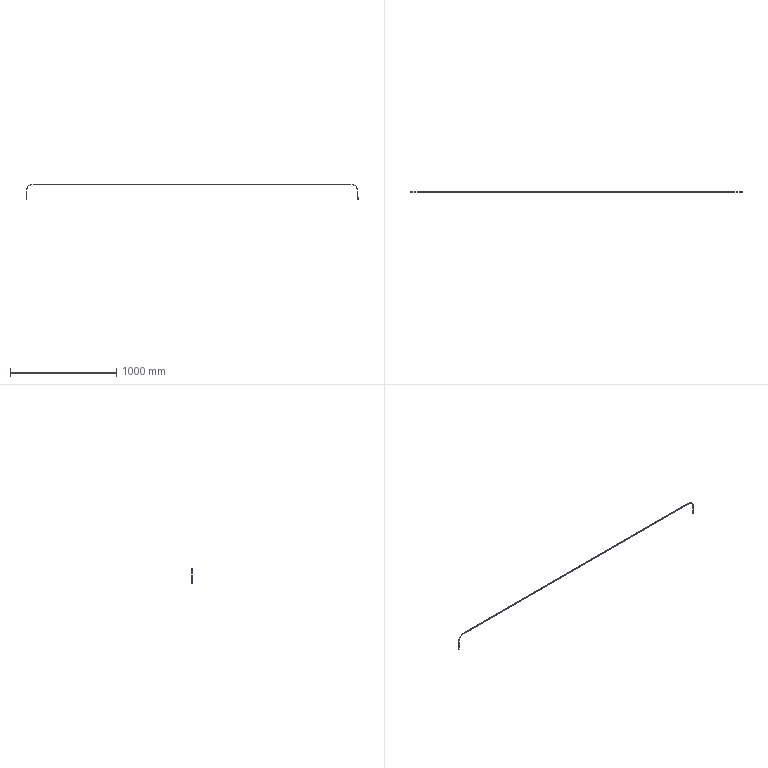Component | SolidWorks | A-SideAluminumCasingAssembly-1_A-SideSealant-1 | 1 solid | 22 faces | box 3131 x 6 x 149.5 mm | volume 60581 mm3 | plane 18 | cylinder 4 | commonest cylinder face diameters 139 x2 133 x2
STEP:
#1=COLOUR_RGB('',0.7922,0.8196,0.9333);
#2=FILL_AREA_STYLE_COLOUR('',#1);
#3=FILL_AREA_STYLE('',(#2));
#4=SURFACE_STYLE_FILL_AREA(#3);
#5=SURFACE_SIDE_STYLE('',(#4));
#6=SURFACE_STYLE_USAGE(.BOTH.,#5);
#7=PRESENTATION_STYLE_ASSIGNMENT((#6));
#8=CARTESIAN_POINT('',(80.551,91.024,73.819));
#9=VERTEX_POINT('',#8);
#10=CARTESIAN_POINT('',(80.551,91.024,73.937));
#11=VERTEX_POINT('',#10);
#12=CARTESIAN_POINT('',(80.551,91.024,73.937));
#13=DIRECTION('',(-0.,0.,1.));
#14=VECTOR('',#13,39.37);
#15=LINE('',#12,#14);
#16=EDGE_CURVE('',#9,#11,#15,.T.);
#17=ORIENTED_EDGE('',*,*,#16,.F.);
#18=CARTESIAN_POINT('',(-37.244,91.024,73.819));
#19=VERTEX_POINT('',#18);
#20=CARTESIAN_POINT('',(-37.244,91.024,73.819));
#21=DIRECTION('',(1.,0.,0.));
#22=VECTOR('',#21,39.37);
#23=LINE('',#20,#22);
#24=EDGE_CURVE('',#19,#9,#23,.T.);
#25=ORIENTED_EDGE('',*,*,#24,.F.);
#26=CARTESIAN_POINT('',(-37.244,91.024,73.937));
#27=VERTEX_POINT('',#26);
#28=CARTESIAN_POINT('',(-37.244,91.024,73.937));
#29=DIRECTION('',(-0.,0.,1.));
#30=VECTOR('',#29,39.37);
#31=LINE('',#28,#30);
#32=EDGE_CURVE('',#19,#27,#31,.T.);
#33=ORIENTED_EDGE('',*,*,#32,.T.);
#34=CARTESIAN_POINT('',(-37.244,91.024,73.937));
#35=DIRECTION('',(1.,0.,0.));
#36=VECTOR('',#35,39.37);
#37=LINE('',#34,#36);
#38=EDGE_CURVE('',#27,#11,#37,.T.);
#39=ORIENTED_EDGE('',*,*,#38,.T.);
#40=EDGE_LOOP('',(#17,#25,#33,#39));
#41=FACE_OUTER_BOUND('',#40,.T.);
#42=CARTESIAN_POINT('',(-37.244,91.024,73.937));
#43=DIRECTION('',(-0.,1.,-0.));
#44=DIRECTION('',(1.,0.,0.));
#45=AXIS2_PLACEMENT_3D('',#42,#43,#44);
#46=PLANE('',#45);
#47=ADVANCED_FACE('',(#41),#46,.T.);
#48=CARTESIAN_POINT('',(-37.244,90.787,73.819));
#49=VERTEX_POINT('',#48);
#50=CARTESIAN_POINT('',(-37.244,90.787,73.937));
#51=VERTEX_POINT('',#50);
#52=CARTESIAN_POINT('',(-37.244,90.787,73.937));
#53=DIRECTION('',(-0.,0.,1.));
#54=VECTOR('',#53,39.37);
#55=LINE('',#52,#54);
#56=EDGE_CURVE('',#49,#51,#55,.T.);
#57=ORIENTED_EDGE('',*,*,#56,.F.);
#58=CARTESIAN_POINT('',(80.551,90.787,73.819));
#59=VERTEX_POINT('',#58);
#60=CARTESIAN_POINT('',(-37.244,90.787,73.819));
#61=DIRECTION('',(1.,0.,0.));
#62=VECTOR('',#61,39.37);
#63=LINE('',#60,#62);
#64=EDGE_CURVE('',#49,#59,#63,.T.);
#65=ORIENTED_EDGE('',*,*,#64,.T.);
#66=CARTESIAN_POINT('',(80.551,90.787,73.937));
#67=VERTEX_POINT('',#66);
#68=CARTESIAN_POINT('',(80.551,90.787,73.937));
#69=DIRECTION('',(-0.,0.,1.));
#70=VECTOR('',#69,39.37);
#71=LINE('',#68,#70);
#72=EDGE_CURVE('',#59,#67,#71,.T.);
#73=ORIENTED_EDGE('',*,*,#72,.T.);
#74=CARTESIAN_POINT('',(-37.244,90.787,73.937));
#75=DIRECTION('',(1.,0.,0.));
#76=VECTOR('',#75,39.37);
#77=LINE('',#74,#76);
#78=EDGE_CURVE('',#51,#67,#77,.T.);
#79=ORIENTED_EDGE('',*,*,#78,.F.);
#80=EDGE_LOOP('',(#57,#65,#73,#79));
#81=FACE_OUTER_BOUND('',#80,.T.);
#82=CARTESIAN_POINT('',(-37.244,90.787,73.937));
#83=DIRECTION('',(-0.,1.,-0.));
#84=DIRECTION('',(1.,0.,0.));
#85=AXIS2_PLACEMENT_3D('',#82,#83,#84);
#86=PLANE('',#85);
#87=ADVANCED_FACE('',(#81),#86,.F.);
#88=ORIENTED_EDGE('',*,*,#78,.T.);
#89=CARTESIAN_POINT('',(80.551,91.024,73.937));
#90=DIRECTION('',(0.,-1.,0.));
#91=VECTOR('',#90,39.37);
#92=LINE('',#89,#91);
#93=EDGE_CURVE('',#11,#67,#92,.T.);
#94=ORIENTED_EDGE('',*,*,#93,.F.);
#95=ORIENTED_EDGE('',*,*,#38,.F.);
#96=CARTESIAN_POINT('',(-37.244,90.787,73.937));
#97=DIRECTION('',(-0.,1.,-0.));
#98=VECTOR('',#97,39.37);
#99=LINE('',#96,#98);
#100=EDGE_CURVE('',#51,#27,#99,.T.);
#101=ORIENTED_EDGE('',*,*,#100,.F.);
#102=EDGE_LOOP('',(#88,#94,#95,#101));
#103=FACE_OUTER_BOUND('',#102,.T.);
#104=CARTESIAN_POINT('',(-37.244,90.787,73.937));
#105=DIRECTION('',(0.,-0.,-1.));
#106=DIRECTION('',(-0.,1.,-0.));
#107=AXIS2_PLACEMENT_3D('',#104,#105,#106);
#108=PLANE('',#107);
#109=ADVANCED_FACE('',(#103),#108,.F.);
#110=ORIENTED_EDGE('',*,*,#64,.F.);
#111=CARTESIAN_POINT('',(-37.244,90.787,73.819));
#112=DIRECTION('',(-0.,1.,-0.));
#113=VECTOR('',#112,39.37);
#114=LINE('',#111,#113);
#115=EDGE_CURVE('',#49,#19,#114,.T.);
#116=ORIENTED_EDGE('',*,*,#115,.T.);
#117=ORIENTED_EDGE('',*,*,#24,.T.);
#118=CARTESIAN_POINT('',(80.551,90.787,73.819));
#119=DIRECTION('',(0.,-1.,0.));
#120=VECTOR('',#119,39.37);
#121=LINE('',#118,#120);
#122=EDGE_CURVE('',#9,#59,#121,.T.);
#123=ORIENTED_EDGE('',*,*,#122,.T.);
#124=EDGE_LOOP('',(#110,#116,#117,#123));
#125=FACE_OUTER_BOUND('',#124,.T.);
#126=CARTESIAN_POINT('',(-37.244,90.787,73.819));
#127=DIRECTION('',(0.,-0.,-1.));
#128=DIRECTION('',(-0.,1.,-0.));
#129=AXIS2_PLACEMENT_3D('',#126,#127,#128);
#130=PLANE('',#129);
#131=ADVANCED_FACE('',(#125),#130,.T.);
#132=CARTESIAN_POINT('',(-39.862,90.787,71.201));
#133=VERTEX_POINT('',#132);
#134=CARTESIAN_POINT('',(-39.98,90.787,71.201));
#135=VERTEX_POINT('',#134);
#136=CARTESIAN_POINT('',(-39.98,90.787,71.201));
#137=DIRECTION('',(-1.,-0.,0.));
#138=VECTOR('',#137,39.37);
#139=LINE('',#136,#138);
#140=EDGE_CURVE('',#133,#135,#139,.T.);
#141=ORIENTED_EDGE('',*,*,#140,.F.);
#142=CARTESIAN_POINT('',(-37.244,90.787,71.201));
#143=DIRECTION('',(0.,-1.,0.));
#144=DIRECTION('',(0.,0.,1.));
#145=AXIS2_PLACEMENT_3D('',#142,#143,#144);
#146=CIRCLE('',#145,2.618);
#147=EDGE_CURVE('',#49,#133,#146,.T.);
#148=ORIENTED_EDGE('',*,*,#147,.F.);
#149=ORIENTED_EDGE('',*,*,#56,.T.);
#150=CARTESIAN_POINT('',(-37.244,90.787,71.201));
#151=DIRECTION('',(0.,-1.,0.));
#152=DIRECTION('',(0.,0.,1.));
#153=AXIS2_PLACEMENT_3D('',#150,#151,#152);
#154=CIRCLE('',#153,2.736);
#155=EDGE_CURVE('',#51,#135,#154,.T.);
#156=ORIENTED_EDGE('',*,*,#155,.T.);
#157=EDGE_LOOP('',(#141,#148,#149,#156));
#158=FACE_OUTER_BOUND('',#157,.T.);
#159=CARTESIAN_POINT('',(-37.244,90.787,71.201));
#160=DIRECTION('',(0.,-1.,0.));
#161=DIRECTION('',(0.,-0.,-1.));
#162=AXIS2_PLACEMENT_3D('',#159,#160,#161);
#163=PLANE('',#162);
#164=ADVANCED_FACE('',(#158),#163,.T.);
#165=CARTESIAN_POINT('',(-39.862,91.024,71.201));
#166=VERTEX_POINT('',#165);
#167=CARTESIAN_POINT('',(-37.244,91.024,71.201));
#168=DIRECTION('',(-0.,1.,-0.));
#169=DIRECTION('',(0.,0.,1.));
#170=AXIS2_PLACEMENT_3D('',#167,#168,#169);
#171=CIRCLE('',#170,2.618);
#172=EDGE_CURVE('',#166,#19,#171,.T.);
#173=ORIENTED_EDGE('',*,*,#172,.F.);
#174=CARTESIAN_POINT('',(-39.98,91.024,71.201));
#175=VERTEX_POINT('',#174);
#176=CARTESIAN_POINT('',(-39.862,91.024,71.201));
#177=DIRECTION('',(-1.,-0.,0.));
#178=VECTOR('',#177,39.37);
#179=LINE('',#176,#178);
#180=EDGE_CURVE('',#166,#175,#179,.T.);
#181=ORIENTED_EDGE('',*,*,#180,.T.);
#182=CARTESIAN_POINT('',(-37.244,91.024,71.201));
#183=DIRECTION('',(-0.,1.,-0.));
#184=DIRECTION('',(0.,0.,1.));
#185=AXIS2_PLACEMENT_3D('',#182,#183,#184);
#186=CIRCLE('',#185,2.736);
#187=EDGE_CURVE('',#175,#27,#186,.T.);
#188=ORIENTED_EDGE('',*,*,#187,.T.);
#189=ORIENTED_EDGE('',*,*,#32,.F.);
#190=EDGE_LOOP('',(#173,#181,#188,#189));
#191=FACE_OUTER_BOUND('',#190,.T.);
#192=CARTESIAN_POINT('',(-37.244,91.024,71.201));
#193=DIRECTION('',(0.,-1.,0.));
#194=DIRECTION('',(0.,-0.,-1.));
#195=AXIS2_PLACEMENT_3D('',#192,#193,#194);
#196=PLANE('',#195);
#197=ADVANCED_FACE('',(#191),#196,.F.);
#198=ORIENTED_EDGE('',*,*,#100,.T.);
#199=ORIENTED_EDGE('',*,*,#187,.F.);
#200=CARTESIAN_POINT('',(-39.98,90.787,71.201));
#201=DIRECTION('',(0.,-1.,0.));
#202=VECTOR('',#201,39.37);
#203=LINE('',#200,#202);
#204=EDGE_CURVE('',#175,#135,#203,.T.);
#205=ORIENTED_EDGE('',*,*,#204,.T.);
#206=ORIENTED_EDGE('',*,*,#155,.F.);
#207=EDGE_LOOP('',(#198,#199,#205,#206));
#208=FACE_OUTER_BOUND('',#207,.T.);
#209=CARTESIAN_POINT('',(-37.244,91.024,71.201));
#210=DIRECTION('',(-0.,1.,-0.));
#211=DIRECTION('',(-1.,-0.,0.));
#212=AXIS2_PLACEMENT_3D('',#209,#210,#211);
#213=CYLINDRICAL_SURFACE('',#212,2.736);
#214=ADVANCED_FACE('',(#208),#213,.T.);
#215=ORIENTED_EDGE('',*,*,#115,.F.);
#216=ORIENTED_EDGE('',*,*,#147,.T.);
#217=CARTESIAN_POINT('',(-39.862,90.787,71.201));
#218=DIRECTION('',(-0.,1.,-0.));
#219=VECTOR('',#218,39.37);
#220=LINE('',#217,#219);
#221=EDGE_CURVE('',#133,#166,#220,.T.);
#222=ORIENTED_EDGE('',*,*,#221,.T.);
#223=ORIENTED_EDGE('',*,*,#172,.T.);
#224=EDGE_LOOP('',(#215,#216,#222,#223));
#225=FACE_OUTER_BOUND('',#224,.T.);
#226=CARTESIAN_POINT('',(-37.244,91.024,71.201));
#227=DIRECTION('',(-0.,1.,-0.));
#228=DIRECTION('',(-1.,-0.,0.));
#229=AXIS2_PLACEMENT_3D('',#226,#227,#228);
#230=CYLINDRICAL_SURFACE('',#229,2.618);
#231=ADVANCED_FACE('',(#225),#230,.F.);
#232=ORIENTED_EDGE('',*,*,#140,.T.);
#233=CARTESIAN_POINT('',(-39.98,90.787,68.051));
#234=VERTEX_POINT('',#233);
#235=CARTESIAN_POINT('',(-39.98,90.787,73.819));
#236=DIRECTION('',(0.,0.,1.));
#237=VECTOR('',#236,39.37);
#238=LINE('',#235,#237);
#239=EDGE_CURVE('',#234,#135,#238,.T.);
#240=ORIENTED_EDGE('',*,*,#239,.F.);
#241=CARTESIAN_POINT('',(-39.862,90.787,68.051));
#242=VERTEX_POINT('',#241);
#243=CARTESIAN_POINT('',(-39.98,90.787,68.051));
#244=DIRECTION('',(1.,0.,-0.));
#245=VECTOR('',#244,39.37);
#246=LINE('',#243,#245);
#247=EDGE_CURVE('',#234,#242,#246,.T.);
#248=ORIENTED_EDGE('',*,*,#247,.T.);
#249=CARTESIAN_POINT('',(-39.862,90.787,73.819));
#250=DIRECTION('',(0.,0.,1.));
#251=VECTOR('',#250,39.37);
#252=LINE('',#249,#251);
#253=EDGE_CURVE('',#242,#133,#252,.T.);
#254=ORIENTED_EDGE('',*,*,#253,.T.);
#255=EDGE_LOOP('',(#232,#240,#248,#254));
#256=FACE_OUTER_BOUND('',#255,.T.);
#257=CARTESIAN_POINT('',(-39.98,90.787,73.819));
#258=DIRECTION('',(-0.,1.,-0.));
#259=DIRECTION('',(-0.,0.,1.));
#260=AXIS2_PLACEMENT_3D('',#257,#258,#259);
#261=PLANE('',#260);
#262=ADVANCED_FACE('',(#256),#261,.F.);
#263=ORIENTED_EDGE('',*,*,#180,.F.);
#264=CARTESIAN_POINT('',(-39.862,91.024,68.051));
#265=VERTEX_POINT('',#264);
#266=CARTESIAN_POINT('',(-39.862,91.024,68.051));
#267=DIRECTION('',(-0.,-0.,-1.));
#268=VECTOR('',#267,39.37);
#269=LINE('',#266,#268);
#270=EDGE_CURVE('',#166,#265,#269,.T.);
#271=ORIENTED_EDGE('',*,*,#270,.T.);
#272=CARTESIAN_POINT('',(-39.98,91.024,68.051));
#273=VERTEX_POINT('',#272);
#274=CARTESIAN_POINT('',(-39.98,91.024,68.051));
#275=DIRECTION('',(1.,0.,-0.));
#276=VECTOR('',#275,39.37);
#277=LINE('',#274,#276);
#278=EDGE_CURVE('',#273,#265,#277,.T.);
#279=ORIENTED_EDGE('',*,*,#278,.F.);
#280=CARTESIAN_POINT('',(-39.98,91.024,73.819));
#281=DIRECTION('',(-0.,-0.,-1.));
#282=VECTOR('',#281,39.37);
#283=LINE('',#280,#282);
#284=EDGE_CURVE('',#175,#273,#283,.T.);
#285=ORIENTED_EDGE('',*,*,#284,.F.);
#286=EDGE_LOOP('',(#263,#271,#279,#285));
#287=FACE_OUTER_BOUND('',#286,.T.);
#288=CARTESIAN_POINT('',(-39.98,91.024,68.051));
#289=DIRECTION('',(0.,-1.,0.));
#290=DIRECTION('',(0.,-0.,-1.));
#291=AXIS2_PLACEMENT_3D('',#288,#289,#290);
#292=PLANE('',#291);
#293=ADVANCED_FACE('',(#287),#292,.F.);
#294=ORIENTED_EDGE('',*,*,#204,.F.);
#295=ORIENTED_EDGE('',*,*,#284,.T.);
#296=CARTESIAN_POINT('',(-39.98,90.787,68.051));
#297=DIRECTION('',(0.,-1.,0.));
#298=VECTOR('',#297,39.37);
#299=LINE('',#296,#298);
#300=EDGE_CURVE('',#273,#234,#299,.T.);
#301=ORIENTED_EDGE('',*,*,#300,.T.);
#302=ORIENTED_EDGE('',*,*,#239,.T.);
#303=EDGE_LOOP('',(#294,#295,#301,#302));
#304=FACE_OUTER_BOUND('',#303,.T.);
#305=CARTESIAN_POINT('',(-39.98,90.787,73.819));
#306=DIRECTION('',(1.,0.,-0.));
#307=DIRECTION('',(0.,0.,1.));
#308=AXIS2_PLACEMENT_3D('',#305,#306,#307);
#309=PLANE('',#308);
#310=ADVANCED_FACE('',(#304),#309,.F.);
#311=ORIENTED_EDGE('',*,*,#270,.F.);
#312=ORIENTED_EDGE('',*,*,#221,.F.);
#313=ORIENTED_EDGE('',*,*,#253,.F.);
#314=CARTESIAN_POINT('',(-39.862,90.787,68.051));
#315=DIRECTION('',(0.,-1.,0.));
#316=VECTOR('',#315,39.37);
#317=LINE('',#314,#316);
#318=EDGE_CURVE('',#265,#242,#317,.T.);
#319=ORIENTED_EDGE('',*,*,#318,.F.);
#320=EDGE_LOOP('',(#311,#312,#313,#319));
#321=FACE_OUTER_BOUND('',#320,.T.);
#322=CARTESIAN_POINT('',(-39.862,90.787,73.819));
#323=DIRECTION('',(1.,0.,-0.));
#324=DIRECTION('',(0.,0.,1.));
#325=AXIS2_PLACEMENT_3D('',#322,#323,#324);
#326=PLANE('',#325);
#327=ADVANCED_FACE('',(#321),#326,.T.);
#328=ORIENTED_EDGE('',*,*,#318,.T.);
#329=ORIENTED_EDGE('',*,*,#247,.F.);
#330=ORIENTED_EDGE('',*,*,#300,.F.);
#331=ORIENTED_EDGE('',*,*,#278,.T.);
#332=EDGE_LOOP('',(#328,#329,#330,#331));
#333=FACE_OUTER_BOUND('',#332,.T.);
#334=CARTESIAN_POINT('',(-39.98,90.787,68.051));
#335=DIRECTION('',(0.,0.,1.));
#336=DIRECTION('',(-1.,-0.,0.));
#337=AXIS2_PLACEMENT_3D('',#334,#335,#336);
#338=PLANE('',#337);
#339=ADVANCED_FACE('',(#333),#338,.F.);
#340=CARTESIAN_POINT('',(83.169,91.024,71.201));
#341=VERTEX_POINT('',#340);
#342=CARTESIAN_POINT('',(83.287,91.024,71.201));
#343=VERTEX_POINT('',#342);
#344=CARTESIAN_POINT('',(83.287,91.024,71.201));
#345=DIRECTION('',(1.,0.,0.));
#346=VECTOR('',#345,39.37);
#347=LINE('',#344,#346);
#348=EDGE_CURVE('',#341,#343,#347,.T.);
#349=ORIENTED_EDGE('',*,*,#348,.F.);
#350=CARTESIAN_POINT('',(80.551,91.024,71.201));
#351=DIRECTION('',(-0.,1.,-0.));
#352=DIRECTION('',(0.,-0.,-1.));
#353=AXIS2_PLACEMENT_3D('',#350,#351,#352);
#354=CIRCLE('',#353,2.618);
#355=EDGE_CURVE('',#9,#341,#354,.T.);
#356=ORIENTED_EDGE('',*,*,#355,.F.);
#357=ORIENTED_EDGE('',*,*,#16,.T.);
#358=CARTESIAN_POINT('',(80.551,91.024,71.201));
#359=DIRECTION('',(-0.,1.,-0.));
#360=DIRECTION('',(0.,-0.,-1.));
#361=AXIS2_PLACEMENT_3D('',#358,#359,#360);
#362=CIRCLE('',#361,2.736);
#363=EDGE_CURVE('',#11,#343,#362,.T.);
#364=ORIENTED_EDGE('',*,*,#363,.T.);
#365=EDGE_LOOP('',(#349,#356,#357,#364));
#366=FACE_OUTER_BOUND('',#365,.T.);
#367=CARTESIAN_POINT('',(80.551,91.024,71.201));
#368=DIRECTION('',(-0.,1.,-0.));
#369=DIRECTION('',(-0.,0.,1.));
#370=AXIS2_PLACEMENT_3D('',#367,#368,#369);
#371=PLANE('',#370);
#372=ADVANCED_FACE('',(#366),#371,.T.);
#373=CARTESIAN_POINT('',(83.169,90.787,71.201));
#374=VERTEX_POINT('',#373);
#375=CARTESIAN_POINT('',(80.551,90.787,71.201));
#376=DIRECTION('',(0.,-1.,0.));
#377=DIRECTION('',(0.,-0.,-1.));
#378=AXIS2_PLACEMENT_3D('',#375,#376,#377);
#379=CIRCLE('',#378,2.618);
#380=EDGE_CURVE('',#374,#59,#379,.T.);
#381=ORIENTED_EDGE('',*,*,#380,.F.);
#382=CARTESIAN_POINT('',(83.287,90.787,71.201));
#383=VERTEX_POINT('',#382);
#384=CARTESIAN_POINT('',(83.169,90.787,71.201));
#385=DIRECTION('',(1.,0.,0.));
#386=VECTOR('',#385,39.37);
#387=LINE('',#384,#386);
#388=EDGE_CURVE('',#374,#383,#387,.T.);
#389=ORIENTED_EDGE('',*,*,#388,.T.);
#390=CARTESIAN_POINT('',(80.551,90.787,71.201));
#391=DIRECTION('',(0.,-1.,0.));
#392=DIRECTION('',(0.,-0.,-1.));
#393=AXIS2_PLACEMENT_3D('',#390,#391,#392);
#394=CIRCLE('',#393,2.736);
#395=EDGE_CURVE('',#383,#67,#394,.T.);
#396=ORIENTED_EDGE('',*,*,#395,.T.);
#397=ORIENTED_EDGE('',*,*,#72,.F.);
#398=EDGE_LOOP('',(#381,#389,#396,#397));
#399=FACE_OUTER_BOUND('',#398,.T.);
#400=CARTESIAN_POINT('',(80.551,90.787,71.201));
#401=DIRECTION('',(-0.,1.,-0.));
#402=DIRECTION('',(-0.,0.,1.));
#403=AXIS2_PLACEMENT_3D('',#400,#401,#402);
#404=PLANE('',#403);
#405=ADVANCED_FACE('',(#399),#404,.F.);
#406=ORIENTED_EDGE('',*,*,#93,.T.);
#407=ORIENTED_EDGE('',*,*,#395,.F.);
#408=CARTESIAN_POINT('',(83.287,91.024,71.201));
#409=DIRECTION('',(-0.,1.,-0.));
#410=VECTOR('',#409,39.37);
#411=LINE('',#408,#410);
#412=EDGE_CURVE('',#383,#343,#411,.T.);
#413=ORIENTED_EDGE('',*,*,#412,.T.);
#414=ORIENTED_EDGE('',*,*,#363,.F.);
#415=EDGE_LOOP('',(#406,#407,#413,#414));
#416=FACE_OUTER_BOUND('',#415,.T.);
#417=CARTESIAN_POINT('',(80.551,90.787,71.201));
#418=DIRECTION('',(0.,-1.,0.));
#419=DIRECTION('',(1.,0.,0.));
#420=AXIS2_PLACEMENT_3D('',#417,#418,#419);
#421=CYLINDRICAL_SURFACE('',#420,2.736);
#422=ADVANCED_FACE('',(#416),#421,.T.);
#423=ORIENTED_EDGE('',*,*,#122,.F.);
#424=ORIENTED_EDGE('',*,*,#355,.T.);
#425=CARTESIAN_POINT('',(83.169,91.024,71.201));
#426=DIRECTION('',(0.,-1.,0.));
#427=VECTOR('',#426,39.37);
#428=LINE('',#425,#427);
#429=EDGE_CURVE('',#341,#374,#428,.T.);
#430=ORIENTED_EDGE('',*,*,#429,.T.);
#431=ORIENTED_EDGE('',*,*,#380,.T.);
#432=EDGE_LOOP('',(#423,#424,#430,#431));
#433=FACE_OUTER_BOUND('',#432,.T.);
#434=CARTESIAN_POINT('',(80.551,90.787,71.201));
#435=DIRECTION('',(0.,-1.,0.));
#436=DIRECTION('',(1.,0.,0.));
#437=AXIS2_PLACEMENT_3D('',#434,#435,#436);
#438=CYLINDRICAL_SURFACE('',#437,2.618);
#439=ADVANCED_FACE('',(#433),#438,.F.);
#440=ORIENTED_EDGE('',*,*,#348,.T.);
#441=CARTESIAN_POINT('',(83.287,91.024,68.051));
#442=VERTEX_POINT('',#441);
#443=CARTESIAN_POINT('',(83.287,91.024,73.819));
#444=DIRECTION('',(-0.,0.,1.));
#445=VECTOR('',#444,39.37);
#446=LINE('',#443,#445);
#447=EDGE_CURVE('',#442,#343,#446,.T.);
#448=ORIENTED_EDGE('',*,*,#447,.F.);
#449=CARTESIAN_POINT('',(83.169,91.024,68.051));
#450=VERTEX_POINT('',#449);
#451=CARTESIAN_POINT('',(83.287,91.024,68.051));
#452=DIRECTION('',(-1.,-0.,-0.));
#453=VECTOR('',#452,39.37);
#454=LINE('',#451,#453);
#455=EDGE_CURVE('',#442,#450,#454,.T.);
#456=ORIENTED_EDGE('',*,*,#455,.T.);
#457=CARTESIAN_POINT('',(83.169,91.024,73.819));
#458=DIRECTION('',(-0.,0.,1.));
#459=VECTOR('',#458,39.37);
#460=LINE('',#457,#459);
#461=EDGE_CURVE('',#450,#341,#460,.T.);
#462=ORIENTED_EDGE('',*,*,#461,.T.);
#463=EDGE_LOOP('',(#440,#448,#456,#462));
#464=FACE_OUTER_BOUND('',#463,.T.);
#465=CARTESIAN_POINT('',(83.287,91.024,73.819));
#466=DIRECTION('',(0.,-1.,0.));
#467=DIRECTION('',(0.,-0.,-1.));
#468=AXIS2_PLACEMENT_3D('',#465,#466,#467);
#469=PLANE('',#468);
#470=ADVANCED_FACE('',(#464),#469,.F.);
#471=ORIENTED_EDGE('',*,*,#388,.F.);
#472=CARTESIAN_POINT('',(83.169,90.787,68.051));
#473=VERTEX_POINT('',#472);
#474=CARTESIAN_POINT('',(83.169,90.787,68.051));
#475=DIRECTION('',(0.,-0.,-1.));
#476=VECTOR('',#475,39.37);
#477=LINE('',#474,#476);
#478=EDGE_CURVE('',#374,#473,#477,.T.);
#479=ORIENTED_EDGE('',*,*,#478,.T.);
#480=CARTESIAN_POINT('',(83.287,90.787,68.051));
#481=VERTEX_POINT('',#480);
#482=CARTESIAN_POINT('',(83.287,90.787,68.051));
#483=DIRECTION('',(-1.,-0.,-0.));
#484=VECTOR('',#483,39.37);
#485=LINE('',#482,#484);
#486=EDGE_CURVE('',#481,#473,#485,.T.);
#487=ORIENTED_EDGE('',*,*,#486,.F.);
#488=CARTESIAN_POINT('',(83.287,90.787,73.819));
#489=DIRECTION('',(0.,-0.,-1.));
#490=VECTOR('',#489,39.37);
#491=LINE('',#488,#490);
#492=EDGE_CURVE('',#383,#481,#491,.T.);
#493=ORIENTED_EDGE('',*,*,#492,.F.);
#494=EDGE_LOOP('',(#471,#479,#487,#493));
#495=FACE_OUTER_BOUND('',#494,.T.);
#496=CARTESIAN_POINT('',(83.287,90.787,68.051));
#497=DIRECTION('',(-0.,1.,-0.));
#498=DIRECTION('',(-0.,0.,1.));
#499=AXIS2_PLACEMENT_3D('',#496,#497,#498);
#500=PLANE('',#499);
#501=ADVANCED_FACE('',(#495),#500,.F.);
#502=ORIENTED_EDGE('',*,*,#412,.F.);
#503=ORIENTED_EDGE('',*,*,#492,.T.);
#504=CARTESIAN_POINT('',(83.287,90.787,68.051));
#505=DIRECTION('',(-0.,1.,-0.));
#506=VECTOR('',#505,39.37);
#507=LINE('',#504,#506);
#508=EDGE_CURVE('',#481,#442,#507,.T.);
#509=ORIENTED_EDGE('',*,*,#508,.T.);
#510=ORIENTED_EDGE('',*,*,#447,.T.);
#511=EDGE_LOOP('',(#502,#503,#509,#510));
#512=FACE_OUTER_BOUND('',#511,.T.);
#513=CARTESIAN_POINT('',(83.287,90.787,73.819));
#514=DIRECTION('',(-1.,-0.,-0.));
#515=DIRECTION('',(0.,-0.,-1.));
#516=AXIS2_PLACEMENT_3D('',#513,#514,#515);
#517=PLANE('',#516);
#518=ADVANCED_FACE('',(#512),#517,.F.);
#519=ORIENTED_EDGE('',*,*,#478,.F.);
#520=ORIENTED_EDGE('',*,*,#429,.F.);
#521=ORIENTED_EDGE('',*,*,#461,.F.);
#522=CARTESIAN_POINT('',(83.169,91.024,68.051));
#523=DIRECTION('',(-0.,1.,-0.));
#524=VECTOR('',#523,39.37);
#525=LINE('',#522,#524);
#526=EDGE_CURVE('',#473,#450,#525,.T.);
#527=ORIENTED_EDGE('',*,*,#526,.F.);
#528=EDGE_LOOP('',(#519,#520,#521,#527));
#529=FACE_OUTER_BOUND('',#528,.T.);
#530=CARTESIAN_POINT('',(83.169,90.787,73.819));
#531=DIRECTION('',(-1.,-0.,-0.));
#532=DIRECTION('',(0.,-0.,-1.));
#533=AXIS2_PLACEMENT_3D('',#530,#531,#532);
#534=PLANE('',#533);
#535=ADVANCED_FACE('',(#529),#534,.T.);
#536=ORIENTED_EDGE('',*,*,#526,.T.);
#537=ORIENTED_EDGE('',*,*,#455,.F.);
#538=ORIENTED_EDGE('',*,*,#508,.F.);
#539=ORIENTED_EDGE('',*,*,#486,.T.);
#540=EDGE_LOOP('',(#536,#537,#538,#539));
#541=FACE_OUTER_BOUND('',#540,.T.);
#542=CARTESIAN_POINT('',(83.287,91.024,68.051));
#543=DIRECTION('',(-0.,0.,1.));
#544=DIRECTION('',(-1.,-0.,-0.));
#545=AXIS2_PLACEMENT_3D('',#542,#543,#544);
#546=PLANE('',#545);
#547=ADVANCED_FACE('',(#541),#546,.F.);
#548=CLOSED_SHELL('',(#47,#87,#109,#131,#164,#197,#214,#231,#262,#293,#310,#327,#339,#372,#405,#422,#439,#470,#501,#518,#535,#547));
#549=MANIFOLD_SOLID_BREP('',#548);
#550=STYLED_ITEM('',(#7),#549);
#551=PRESENTATION_LAYER_ASSIGNMENT('','',(#550));
#552=CARTESIAN_POINT('',(0.,0.,0.));
#553=DIRECTION('',(0.,0.,1.));
#554=DIRECTION('',(1.,0.,0.));
#555=AXIS2_PLACEMENT_3D('',#552,#553,#554);
#556=(LENGTH_UNIT()NAMED_UNIT(*)SI_UNIT($,.METRE.));
#557=LENGTH_MEASURE_WITH_UNIT(LENGTH_MEASURE(0.0254),#556);
#558=DIMENSIONAL_EXPONENTS(1.,0.,0.,0.,0.,0.,0.);
#559=(CONVERSION_BASED_UNIT('',#557)LENGTH_UNIT()NAMED_UNIT(#558));
#560=UNCERTAINTY_MEASURE_WITH_UNIT(LENGTH_MEASURE(0.00001),#559,'','');
#561=(NAMED_UNIT(*)PLANE_ANGLE_UNIT()SI_UNIT($,.RADIAN.));
#562=(NAMED_UNIT(*)SI_UNIT($,.STERADIAN.)SOLID_ANGLE_UNIT());
#563=(GEOMETRIC_REPRESENTATION_CONTEXT(3)GLOBAL_UNCERTAINTY_ASSIGNED_CONTEXT((#560))GLOBAL_UNIT_ASSIGNED_CONTEXT((#559,#561,#562))REPRESENTATION_CONTEXT('',''));
#564=ADVANCED_BREP_SHAPE_REPRESENTATION('',(#549,#555),#563);
#565=(LENGTH_UNIT()NAMED_UNIT(*)SI_UNIT($,.METRE.));
#566=LENGTH_MEASURE_WITH_UNIT(LENGTH_MEASURE(0.0254),#565);
#567=DIMENSIONAL_EXPONENTS(1.,0.,0.,0.,0.,0.,0.);
#568=(CONVERSION_BASED_UNIT('',#566)LENGTH_UNIT()NAMED_UNIT(#567));
#569=UNCERTAINTY_MEASURE_WITH_UNIT(LENGTH_MEASURE(0.00001),#568,'','');
#570=(NAMED_UNIT(*)PLANE_ANGLE_UNIT()SI_UNIT($,.RADIAN.));
#571=(NAMED_UNIT(*)SI_UNIT($,.STERADIAN.)SOLID_ANGLE_UNIT());
#572=(GEOMETRIC_REPRESENTATION_CONTEXT(3)GLOBAL_UNCERTAINTY_ASSIGNED_CONTEXT((#569))GLOBAL_UNIT_ASSIGNED_CONTEXT((#568,#570,#571))REPRESENTATION_CONTEXT('',''));
#573=MECHANICAL_DESIGN_GEOMETRIC_PRESENTATION_REPRESENTATION('',(#550),#572);